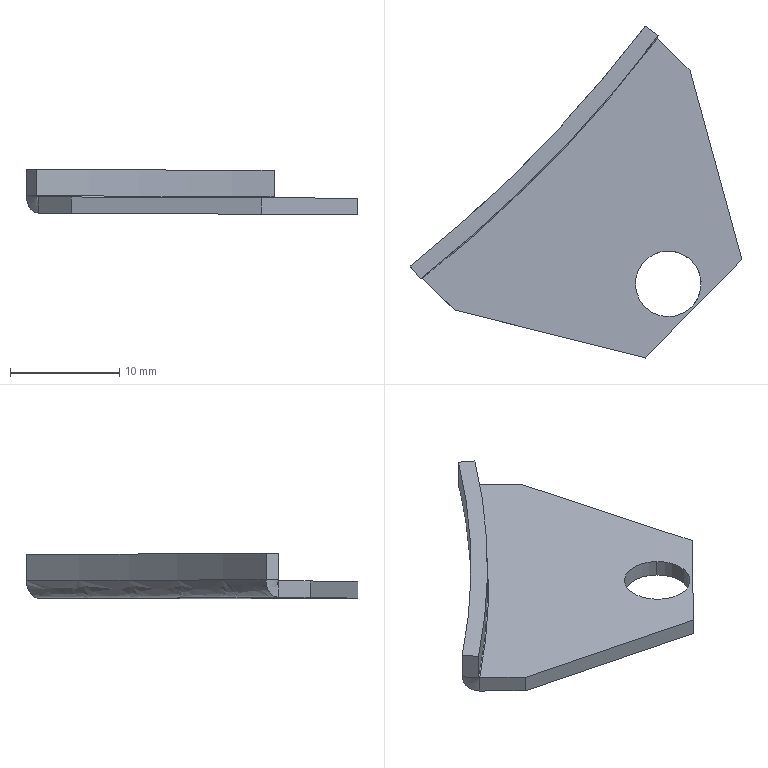Component | SolidWorks | Light-1_LampHolderMountingPlate-11 | 1 solid | 18 faces | box 30.32 x 30.33 x 4.13 mm | volume 795 mm3 | plane 10 | cylinder 4 | spline 4 | commonest cylinder face diameters 6 x2 244.197 x1 247.197 x1
STEP:
#1=CARTESIAN_POINT('',(-209.83,272.853,13.52));
#2=VERTEX_POINT('',#1);
#3=CARTESIAN_POINT('',(-209.665,273.022,13.52));
#4=VERTEX_POINT('',#3);
#5=CARTESIAN_POINT('',(-209.748,272.937,13.52));
#6=DIRECTION('',(0.004294,0.,1.));
#7=DIRECTION('',(-0.6995,-0.7146,0.003003));
#8=AXIS2_PLACEMENT_3D('',#5,#6,#7);
#9=CIRCLE('',#8,0.1181);
#10=EDGE_CURVE('',#2,#4,#9,.T.);
#11=ORIENTED_EDGE('',*,*,#10,.T.);
#12=CARTESIAN_POINT('',(-209.665,273.022,13.461));
#13=VERTEX_POINT('',#12);
#14=CARTESIAN_POINT('',(-209.665,273.022,13.52));
#15=DIRECTION('',(-0.004294,-0.,-1.));
#16=VECTOR('',#15,39.37);
#17=LINE('',#14,#16);
#18=EDGE_CURVE('',#4,#13,#17,.T.);
#19=ORIENTED_EDGE('',*,*,#18,.T.);
#20=CARTESIAN_POINT('',(-209.83,272.853,13.461));
#21=VERTEX_POINT('',#20);
#22=CARTESIAN_POINT('',(-209.748,272.937,13.461));
#23=DIRECTION('',(-0.004294,-0.,-1.));
#24=DIRECTION('',(-0.6995,-0.7146,0.003003));
#25=AXIS2_PLACEMENT_3D('',#22,#23,#24);
#26=CIRCLE('',#25,0.1181);
#27=EDGE_CURVE('',#13,#21,#26,.T.);
#28=ORIENTED_EDGE('',*,*,#27,.T.);
#29=CARTESIAN_POINT('',(-209.83,272.853,13.52));
#30=DIRECTION('',(-0.004294,-0.,-1.));
#31=VECTOR('',#30,39.37);
#32=LINE('',#29,#31);
#33=EDGE_CURVE('',#2,#21,#32,.T.);
#34=ORIENTED_EDGE('',*,*,#33,.F.);
#35=EDGE_LOOP('',(#11,#19,#28,#34));
#36=FACE_OUTER_BOUND('',#35,.T.);
#37=CARTESIAN_POINT('',(-209.748,272.937,13.52));
#38=DIRECTION('',(-0.004294,-0.,-1.));
#39=DIRECTION('',(-0.6995,-0.7146,0.003003));
#40=AXIS2_PLACEMENT_3D('',#37,#38,#39);
#41=CYLINDRICAL_SURFACE('',#40,0.1181);
#42=ADVANCED_FACE('',(#36),#41,.F.);
#43=ORIENTED_EDGE('',*,*,#18,.F.);
#44=CARTESIAN_POINT('',(-209.748,272.937,13.52));
#45=DIRECTION('',(0.004294,0.,1.));
#46=DIRECTION('',(-0.6995,-0.7146,0.003003));
#47=AXIS2_PLACEMENT_3D('',#44,#45,#46);
#48=CIRCLE('',#47,0.1181);
#49=EDGE_CURVE('',#4,#2,#48,.T.);
#50=ORIENTED_EDGE('',*,*,#49,.T.);
#51=ORIENTED_EDGE('',*,*,#33,.T.);
#52=CARTESIAN_POINT('',(-209.748,272.937,13.461));
#53=DIRECTION('',(-0.004294,-0.,-1.));
#54=DIRECTION('',(-0.6995,-0.7146,0.003003));
#55=AXIS2_PLACEMENT_3D('',#52,#53,#54);
#56=CIRCLE('',#55,0.1181);
#57=EDGE_CURVE('',#21,#13,#56,.T.);
#58=ORIENTED_EDGE('',*,*,#57,.T.);
#59=EDGE_LOOP('',(#43,#50,#51,#58));
#60=FACE_OUTER_BOUND('',#59,.T.);
#61=CARTESIAN_POINT('',(-209.748,272.937,13.52));
#62=DIRECTION('',(-0.004294,-0.,-1.));
#63=DIRECTION('',(-0.6995,-0.7146,0.003003));
#64=AXIS2_PLACEMENT_3D('',#61,#62,#63);
#65=CYLINDRICAL_SURFACE('',#64,0.1181);
#66=ADVANCED_FACE('',(#60),#65,.F.);
#67=ORIENTED_EDGE('',*,*,#57,.F.);
#68=ORIENTED_EDGE('',*,*,#27,.F.);
#69=EDGE_LOOP('',(#67,#68));
#70=FACE_BOUND('',#69,.T.);
#71=CARTESIAN_POINT('',(-209.483,273.025,13.46));
#72=VERTEX_POINT('',#71);
#73=CARTESIAN_POINT('',(-209.83,272.671,13.461));
#74=VERTEX_POINT('',#73);
#75=CARTESIAN_POINT('',(-209.657,272.848,13.461));
#76=DIRECTION('',(-0.6995,-0.7146,0.003003));
#77=VECTOR('',#76,39.37);
#78=LINE('',#75,#77);
#79=EDGE_CURVE('',#72,#74,#78,.T.);
#80=ORIENTED_EDGE('',*,*,#79,.T.);
#81=CARTESIAN_POINT('',(-210.515,272.843,13.464));
#82=VERTEX_POINT('',#81);
#83=CARTESIAN_POINT('',(-209.83,272.671,13.461));
#84=DIRECTION('',(-0.9698,0.2438,0.004164));
#85=VECTOR('',#84,39.37);
#86=LINE('',#83,#85);
#87=EDGE_CURVE('',#74,#82,#86,.T.);
#88=ORIENTED_EDGE('',*,*,#87,.T.);
#89=CARTESIAN_POINT('',(-210.631,272.957,13.465));
#90=VERTEX_POINT('',#89);
#91=CARTESIAN_POINT('',(-210.357,272.688,13.464));
#92=DIRECTION('',(-0.7146,0.6995,0.003068));
#93=VECTOR('',#92,39.37);
#94=LINE('',#91,#93);
#95=EDGE_CURVE('',#82,#90,#94,.T.);
#96=ORIENTED_EDGE('',*,*,#95,.T.);
#97=CARTESIAN_POINT('',(-209.786,273.82,13.461));
#98=VERTEX_POINT('',#97);
#99=CARTESIAN_POINT('',(-210.631,272.957,13.465));
#100=CARTESIAN_POINT('',(-210.592,272.988,13.465));
#101=CARTESIAN_POINT('',(-210.553,273.02,13.465));
#102=CARTESIAN_POINT('',(-210.476,273.086,13.464));
#103=CARTESIAN_POINT('',(-210.438,273.119,13.464));
#104=CARTESIAN_POINT('',(-210.326,273.22,13.464));
#105=CARTESIAN_POINT('',(-210.253,273.29,13.463));
#106=CARTESIAN_POINT('',(-210.147,273.399,13.463));
#107=CARTESIAN_POINT('',(-210.095,273.453,13.463));
#108=CARTESIAN_POINT('',(-210.044,273.51,13.462));
#109=CARTESIAN_POINT('',(-210.01,273.547,13.462));
#110=CARTESIAN_POINT('',(-209.993,273.566,13.462));
#111=CARTESIAN_POINT('',(-209.911,273.662,13.462));
#112=CARTESIAN_POINT('',(-209.847,273.74,13.461));
#113=CARTESIAN_POINT('',(-209.786,273.82,13.461));
#114=B_SPLINE_CURVE_WITH_KNOTS('',3,(#99,#100,#101,#102,#103,#104,#105,#106,#107,#108,#109,#110,#111,#112,#113),.UNSPECIFIED.,.F.,.F.,(4,2,2,2,1,2,2,4),(0.,0.125,0.25,0.5,0.625,0.6875,0.75,1.),.UNSPECIFIED.);
#115=EDGE_CURVE('',#90,#98,#114,.T.);
#116=ORIENTED_EDGE('',*,*,#115,.T.);
#117=CARTESIAN_POINT('',(-209.67,273.706,13.461));
#118=VERTEX_POINT('',#117);
#119=CARTESIAN_POINT('',(-209.512,273.552,13.46));
#120=DIRECTION('',(0.7146,-0.6995,-0.003068));
#121=VECTOR('',#120,39.37);
#122=LINE('',#119,#121);
#123=EDGE_CURVE('',#98,#118,#122,.T.);
#124=ORIENTED_EDGE('',*,*,#123,.T.);
#125=CARTESIAN_POINT('',(-209.67,273.706,13.461));
#126=DIRECTION('',(0.2645,-0.9644,-0.001136));
#127=VECTOR('',#126,39.37);
#128=LINE('',#125,#127);
#129=EDGE_CURVE('',#118,#72,#128,.T.);
#130=ORIENTED_EDGE('',*,*,#129,.T.);
#131=EDGE_LOOP('',(#80,#88,#96,#116,#124,#130));
#132=FACE_OUTER_BOUND('',#131,.T.);
#133=CARTESIAN_POINT('',(-209.234,273.28,13.459));
#134=DIRECTION('',(-0.004294,-0.,-1.));
#135=DIRECTION('',(-0.6995,-0.7146,0.003003));
#136=AXIS2_PLACEMENT_3D('',#133,#134,#135);
#137=PLANE('',#136);
#138=ADVANCED_FACE('',(#70,#132),#137,.T.);
#139=ORIENTED_EDGE('',*,*,#10,.F.);
#140=ORIENTED_EDGE('',*,*,#49,.F.);
#141=EDGE_LOOP('',(#139,#140));
#142=FACE_BOUND('',#141,.T.);
#143=CARTESIAN_POINT('',(-210.514,272.843,13.523));
#144=VERTEX_POINT('',#143);
#145=CARTESIAN_POINT('',(-210.631,272.957,13.524));
#146=VERTEX_POINT('',#145);
#147=CARTESIAN_POINT('',(-210.357,272.688,13.523));
#148=DIRECTION('',(-0.7146,0.6995,0.003068));
#149=VECTOR('',#148,39.37);
#150=LINE('',#147,#149);
#151=EDGE_CURVE('',#144,#146,#150,.T.);
#152=ORIENTED_EDGE('',*,*,#151,.F.);
#153=CARTESIAN_POINT('',(-209.83,272.671,13.52));
#154=VERTEX_POINT('',#153);
#155=CARTESIAN_POINT('',(-209.83,272.671,13.52));
#156=DIRECTION('',(-0.9698,0.2438,0.004164));
#157=VECTOR('',#156,39.37);
#158=LINE('',#155,#157);
#159=EDGE_CURVE('',#154,#144,#158,.T.);
#160=ORIENTED_EDGE('',*,*,#159,.F.);
#161=CARTESIAN_POINT('',(-209.483,273.025,13.519));
#162=VERTEX_POINT('',#161);
#163=CARTESIAN_POINT('',(-209.656,272.848,13.52));
#164=DIRECTION('',(-0.6995,-0.7146,0.003003));
#165=VECTOR('',#164,39.37);
#166=LINE('',#163,#165);
#167=EDGE_CURVE('',#162,#154,#166,.T.);
#168=ORIENTED_EDGE('',*,*,#167,.F.);
#169=CARTESIAN_POINT('',(-209.669,273.706,13.52));
#170=VERTEX_POINT('',#169);
#171=CARTESIAN_POINT('',(-209.669,273.706,13.52));
#172=DIRECTION('',(0.2645,-0.9644,-0.001136));
#173=VECTOR('',#172,39.37);
#174=LINE('',#171,#173);
#175=EDGE_CURVE('',#170,#162,#174,.T.);
#176=ORIENTED_EDGE('',*,*,#175,.F.);
#177=CARTESIAN_POINT('',(-209.786,273.82,13.52));
#178=VERTEX_POINT('',#177);
#179=CARTESIAN_POINT('',(-209.512,273.552,13.519));
#180=DIRECTION('',(0.7146,-0.6995,-0.003068));
#181=VECTOR('',#180,39.37);
#182=LINE('',#179,#181);
#183=EDGE_CURVE('',#178,#170,#182,.T.);
#184=ORIENTED_EDGE('',*,*,#183,.F.);
#185=CARTESIAN_POINT('',(-210.631,272.957,13.524));
#186=CARTESIAN_POINT('',(-210.314,273.209,13.523));
#187=CARTESIAN_POINT('',(-210.031,273.498,13.521));
#188=CARTESIAN_POINT('',(-209.786,273.82,13.52));
#189=(BOUNDED_CURVE()B_SPLINE_CURVE(3,(#185,#186,#187,#188),.UNSPECIFIED.,.F.,.F.)B_SPLINE_CURVE_WITH_KNOTS((4,4),(0.,1.),.UNSPECIFIED.)CURVE()GEOMETRIC_REPRESENTATION_ITEM()RATIONAL_B_SPLINE_CURVE((0.9564,0.9515,0.9515,0.9564))REPRESENTATION_ITEM(''));
#190=EDGE_CURVE('',#146,#178,#189,.T.);
#191=ORIENTED_EDGE('',*,*,#190,.F.);
#192=EDGE_LOOP('',(#152,#160,#168,#176,#184,#191));
#193=FACE_OUTER_BOUND('',#192,.T.);
#194=CARTESIAN_POINT('',(-209.234,273.28,13.518));
#195=DIRECTION('',(-0.004294,-0.,-1.));
#196=DIRECTION('',(-0.6995,-0.7146,0.003003));
#197=AXIS2_PLACEMENT_3D('',#194,#195,#196);
#198=PLANE('',#197);
#199=ADVANCED_FACE('',(#142,#193),#198,.F.);
#200=CARTESIAN_POINT('',(-210.515,272.843,13.494));
#201=DIRECTION('',(-0.004294,-0.,-1.));
#202=VECTOR('',#201,39.37);
#203=LINE('',#200,#202);
#204=EDGE_CURVE('',#144,#82,#203,.T.);
#205=ORIENTED_EDGE('',*,*,#204,.T.);
#206=ORIENTED_EDGE('',*,*,#87,.F.);
#207=CARTESIAN_POINT('',(-209.83,272.671,13.491));
#208=DIRECTION('',(0.004294,0.,1.));
#209=VECTOR('',#208,39.37);
#210=LINE('',#207,#209);
#211=EDGE_CURVE('',#74,#154,#210,.T.);
#212=ORIENTED_EDGE('',*,*,#211,.T.);
#213=ORIENTED_EDGE('',*,*,#159,.T.);
#214=EDGE_LOOP('',(#205,#206,#212,#213));
#215=FACE_OUTER_BOUND('',#214,.T.);
#216=CARTESIAN_POINT('',(-209.83,272.671,13.52));
#217=DIRECTION('',(-0.2438,-0.9698,0.001047));
#218=DIRECTION('',(-0.9698,0.2438,0.004164));
#219=AXIS2_PLACEMENT_3D('',#216,#217,#218);
#220=PLANE('',#219);
#221=ADVANCED_FACE('',(#215),#220,.T.);
#222=ORIENTED_EDGE('',*,*,#79,.F.);
#223=CARTESIAN_POINT('',(-209.483,273.025,13.489));
#224=DIRECTION('',(0.004294,0.,1.));
#225=VECTOR('',#224,39.37);
#226=LINE('',#223,#225);
#227=EDGE_CURVE('',#72,#162,#226,.T.);
#228=ORIENTED_EDGE('',*,*,#227,.T.);
#229=ORIENTED_EDGE('',*,*,#167,.T.);
#230=ORIENTED_EDGE('',*,*,#211,.F.);
#231=EDGE_LOOP('',(#222,#228,#229,#230));
#232=FACE_OUTER_BOUND('',#231,.T.);
#233=CARTESIAN_POINT('',(-209.483,273.025,13.519));
#234=DIRECTION('',(0.7146,-0.6995,-0.003068));
#235=DIRECTION('',(-0.6995,-0.7146,0.003003));
#236=AXIS2_PLACEMENT_3D('',#233,#234,#235);
#237=PLANE('',#236);
#238=ADVANCED_FACE('',(#232),#237,.T.);
#239=ORIENTED_EDGE('',*,*,#227,.F.);
#240=ORIENTED_EDGE('',*,*,#129,.F.);
#241=CARTESIAN_POINT('',(-209.67,273.706,13.49));
#242=DIRECTION('',(0.004294,0.,1.));
#243=VECTOR('',#242,39.37);
#244=LINE('',#241,#243);
#245=EDGE_CURVE('',#118,#170,#244,.T.);
#246=ORIENTED_EDGE('',*,*,#245,.T.);
#247=ORIENTED_EDGE('',*,*,#175,.T.);
#248=EDGE_LOOP('',(#239,#240,#246,#247));
#249=FACE_OUTER_BOUND('',#248,.T.);
#250=CARTESIAN_POINT('',(-209.669,273.706,13.52));
#251=DIRECTION('',(0.9644,0.2645,-0.004141));
#252=DIRECTION('',(0.2645,-0.9644,-0.001136));
#253=AXIS2_PLACEMENT_3D('',#250,#251,#252);
#254=PLANE('',#253);
#255=ADVANCED_FACE('',(#249),#254,.T.);
#256=ORIENTED_EDGE('',*,*,#245,.F.);
#257=ORIENTED_EDGE('',*,*,#123,.F.);
#258=CARTESIAN_POINT('',(-209.786,273.82,13.491));
#259=DIRECTION('',(-0.004294,-0.,-1.));
#260=VECTOR('',#259,39.37);
#261=LINE('',#258,#260);
#262=EDGE_CURVE('',#178,#98,#261,.T.);
#263=ORIENTED_EDGE('',*,*,#262,.F.);
#264=ORIENTED_EDGE('',*,*,#183,.T.);
#265=EDGE_LOOP('',(#256,#257,#263,#264));
#266=FACE_OUTER_BOUND('',#265,.T.);
#267=CARTESIAN_POINT('',(-209.786,273.82,13.52));
#268=DIRECTION('',(0.6995,0.7146,-0.003003));
#269=DIRECTION('',(0.7146,-0.6995,-0.003068));
#270=AXIS2_PLACEMENT_3D('',#267,#268,#269);
#271=PLANE('',#270);
#272=ADVANCED_FACE('',(#266),#271,.T.);
#273=ORIENTED_EDGE('',*,*,#115,.F.);
#274=CARTESIAN_POINT('',(-210.677,273.001,13.528));
#275=VERTEX_POINT('',#274);
#276=CARTESIAN_POINT('',(-210.631,272.957,13.465));
#277=CARTESIAN_POINT('',(-210.634,272.96,13.465));
#278=CARTESIAN_POINT('',(-210.637,272.963,13.465));
#279=CARTESIAN_POINT('',(-210.643,272.969,13.467));
#280=CARTESIAN_POINT('',(-210.645,272.972,13.468));
#281=CARTESIAN_POINT('',(-210.651,272.978,13.471));
#282=CARTESIAN_POINT('',(-210.653,272.98,13.473));
#283=CARTESIAN_POINT('',(-210.658,272.985,13.478));
#284=CARTESIAN_POINT('',(-210.66,272.987,13.481));
#285=CARTESIAN_POINT('',(-210.666,272.994,13.489));
#286=CARTESIAN_POINT('',(-210.67,272.997,13.496));
#287=CARTESIAN_POINT('',(-210.675,273.001,13.511));
#288=CARTESIAN_POINT('',(-210.676,273.002,13.52));
#289=CARTESIAN_POINT('',(-210.677,273.001,13.528));
#290=B_SPLINE_CURVE_WITH_KNOTS('',3,(#276,#277,#278,#279,#280,#281,#282,#283,#284,#285,#286,#287,#288,#289),.UNSPECIFIED.,.F.,.F.,(4,2,2,2,2,2,4),(0.,0.0003134,0.0006269,0.0009403,0.001254,0.001881,0.002507),.UNSPECIFIED.);
#291=EDGE_CURVE('',#90,#275,#290,.T.);
#292=ORIENTED_EDGE('',*,*,#291,.T.);
#293=CARTESIAN_POINT('',(-209.832,273.865,13.524));
#294=VERTEX_POINT('',#293);
#295=CARTESIAN_POINT('',(-213.662,276.769,13.541));
#296=DIRECTION('',(0.004294,0.,1.));
#297=DIRECTION('',(0.6199,-0.7847,-0.002662));
#298=AXIS2_PLACEMENT_3D('',#295,#296,#297);
#299=CIRCLE('',#298,4.807);
#300=EDGE_CURVE('',#275,#294,#299,.T.);
#301=ORIENTED_EDGE('',*,*,#300,.T.);
#302=CARTESIAN_POINT('',(-209.832,273.865,13.524));
#303=CARTESIAN_POINT('',(-209.832,273.865,13.52));
#304=CARTESIAN_POINT('',(-209.832,273.864,13.516));
#305=CARTESIAN_POINT('',(-209.831,273.863,13.508));
#306=CARTESIAN_POINT('',(-209.83,273.862,13.504));
#307=CARTESIAN_POINT('',(-209.828,273.859,13.496));
#308=CARTESIAN_POINT('',(-209.827,273.858,13.493));
#309=CARTESIAN_POINT('',(-209.823,273.854,13.486));
#310=CARTESIAN_POINT('',(-209.821,273.853,13.483));
#311=CARTESIAN_POINT('',(-209.815,273.846,13.474));
#312=CARTESIAN_POINT('',(-209.81,273.842,13.469));
#313=CARTESIAN_POINT('',(-209.799,273.831,13.463));
#314=CARTESIAN_POINT('',(-209.793,273.826,13.461));
#315=CARTESIAN_POINT('',(-209.786,273.82,13.461));
#316=B_SPLINE_CURVE_WITH_KNOTS('',3,(#302,#303,#304,#305,#306,#307,#308,#309,#310,#311,#312,#313,#314,#315),.UNSPECIFIED.,.F.,.F.,(4,2,2,2,2,2,4),(0.,0.0003134,0.0006269,0.0009403,0.001254,0.001881,0.002507),.UNSPECIFIED.);
#317=EDGE_CURVE('',#294,#98,#316,.T.);
#318=ORIENTED_EDGE('',*,*,#317,.T.);
#319=EDGE_LOOP('',(#273,#292,#301,#318));
#320=FACE_OUTER_BOUND('',#319,.T.);
#321=CARTESIAN_POINT('',(-210.64,272.943,13.465));
#322=CARTESIAN_POINT('',(-210.313,273.2,13.464));
#323=CARTESIAN_POINT('',(-210.023,273.497,13.463));
#324=CARTESIAN_POINT('',(-209.772,273.829,13.461));
#325=CARTESIAN_POINT('',(-210.666,272.976,13.461));
#326=CARTESIAN_POINT('',(-210.343,273.232,13.46));
#327=CARTESIAN_POINT('',(-210.055,273.526,13.458));
#328=CARTESIAN_POINT('',(-209.806,273.855,13.457));
#329=CARTESIAN_POINT('',(-210.685,273.,13.492));
#330=CARTESIAN_POINT('',(-210.364,273.254,13.49));
#331=CARTESIAN_POINT('',(-210.077,273.546,13.489));
#332=CARTESIAN_POINT('',(-209.83,273.873,13.488));
#333=CARTESIAN_POINT('',(-210.682,272.997,13.534));
#334=CARTESIAN_POINT('',(-210.361,273.251,13.533));
#335=CARTESIAN_POINT('',(-210.074,273.544,13.532));
#336=CARTESIAN_POINT('',(-209.827,273.87,13.531));
#337=(BOUNDED_SURFACE()B_SPLINE_SURFACE(3,3,((#321,#322,#323,#324),(#325,#326,#327,#328),(#329,#330,#331,#332),(#333,#334,#335,#336)),.UNSPECIFIED.,.F.,.F.,.T.)B_SPLINE_SURFACE_WITH_KNOTS((4,4),(4,4),(0.,1.),(0.,1.),.UNSPECIFIED.)GEOMETRIC_REPRESENTATION_ITEM()RATIONAL_B_SPLINE_SURFACE(((1.,0.9946,0.9946,1.),(0.7553,0.7512,0.7512,0.7553),(0.7553,0.7512,0.7512,0.7553),(1.,0.9946,0.9946,1.)))REPRESENTATION_ITEM('')SURFACE());
#338=ADVANCED_FACE('',(#320),#337,.T.);
#339=ORIENTED_EDGE('',*,*,#95,.F.);
#340=ORIENTED_EDGE('',*,*,#204,.F.);
#341=ORIENTED_EDGE('',*,*,#151,.T.);
#342=CARTESIAN_POINT('',(-210.631,272.957,13.494));
#343=DIRECTION('',(-0.004294,-0.,-1.));
#344=VECTOR('',#343,39.37);
#345=LINE('',#342,#344);
#346=EDGE_CURVE('',#146,#90,#345,.T.);
#347=ORIENTED_EDGE('',*,*,#346,.T.);
#348=EDGE_LOOP('',(#339,#340,#341,#347));
#349=FACE_OUTER_BOUND('',#348,.T.);
#350=CARTESIAN_POINT('',(-210.514,272.843,13.523));
#351=DIRECTION('',(-0.6995,-0.7146,0.003003));
#352=DIRECTION('',(-0.7146,0.6995,0.003068));
#353=AXIS2_PLACEMENT_3D('',#350,#351,#352);
#354=PLANE('',#353);
#355=ADVANCED_FACE('',(#349),#354,.T.);
#356=CARTESIAN_POINT('',(-210.64,272.955,13.528));
#357=VERTEX_POINT('',#356);
#358=CARTESIAN_POINT('',(-210.631,272.957,13.524));
#359=CARTESIAN_POINT('',(-210.633,272.957,13.524));
#360=CARTESIAN_POINT('',(-210.635,272.957,13.524));
#361=CARTESIAN_POINT('',(-210.638,272.956,13.526));
#362=CARTESIAN_POINT('',(-210.639,272.956,13.527));
#363=CARTESIAN_POINT('',(-210.64,272.955,13.528));
#364=B_SPLINE_CURVE_WITH_KNOTS('',3,(#358,#359,#360,#361,#362,#363),.UNSPECIFIED.,.F.,.F.,(4,2,4),(0.,0.0001276,0.0002551),.UNSPECIFIED.);
#365=EDGE_CURVE('',#146,#357,#364,.T.);
#366=ORIENTED_EDGE('',*,*,#365,.F.);
#367=ORIENTED_EDGE('',*,*,#190,.T.);
#368=CARTESIAN_POINT('',(-209.784,273.829,13.524));
#369=VERTEX_POINT('',#368);
#370=CARTESIAN_POINT('',(-209.784,273.829,13.524));
#371=CARTESIAN_POINT('',(-209.785,273.828,13.523));
#372=CARTESIAN_POINT('',(-209.786,273.827,13.522));
#373=CARTESIAN_POINT('',(-209.786,273.824,13.521));
#374=CARTESIAN_POINT('',(-209.786,273.822,13.52));
#375=CARTESIAN_POINT('',(-209.786,273.82,13.52));
#376=B_SPLINE_CURVE_WITH_KNOTS('',3,(#370,#371,#372,#373,#374,#375),.UNSPECIFIED.,.F.,.F.,(4,2,4),(0.,0.0001275,0.0002551),.UNSPECIFIED.);
#377=EDGE_CURVE('',#369,#178,#376,.T.);
#378=ORIENTED_EDGE('',*,*,#377,.F.);
#379=CARTESIAN_POINT('',(-213.662,276.769,13.541));
#380=DIRECTION('',(0.004294,0.,1.));
#381=DIRECTION('',(0.6199,-0.7847,-0.002662));
#382=AXIS2_PLACEMENT_3D('',#379,#380,#381);
#383=CIRCLE('',#382,4.866);
#384=EDGE_CURVE('',#357,#369,#383,.T.);
#385=ORIENTED_EDGE('',*,*,#384,.F.);
#386=EDGE_LOOP('',(#366,#367,#378,#385));
#387=FACE_OUTER_BOUND('',#386,.T.);
#388=CARTESIAN_POINT('',(-210.643,272.947,13.524));
#389=CARTESIAN_POINT('',(-210.317,273.205,13.523));
#390=CARTESIAN_POINT('',(-210.027,273.501,13.521));
#391=CARTESIAN_POINT('',(-209.777,273.832,13.52));
#392=CARTESIAN_POINT('',(-210.645,272.949,13.524));
#393=CARTESIAN_POINT('',(-210.319,273.206,13.522));
#394=CARTESIAN_POINT('',(-210.029,273.503,13.521));
#395=CARTESIAN_POINT('',(-209.779,273.834,13.52));
#396=CARTESIAN_POINT('',(-210.646,272.951,13.526));
#397=CARTESIAN_POINT('',(-210.32,273.208,13.524));
#398=CARTESIAN_POINT('',(-210.03,273.504,13.523));
#399=CARTESIAN_POINT('',(-209.78,273.835,13.522));
#400=CARTESIAN_POINT('',(-210.646,272.951,13.528));
#401=CARTESIAN_POINT('',(-210.32,273.208,13.527));
#402=CARTESIAN_POINT('',(-210.03,273.504,13.526));
#403=CARTESIAN_POINT('',(-209.78,273.835,13.525));
#404=(BOUNDED_SURFACE()B_SPLINE_SURFACE(3,3,((#388,#389,#390,#391),(#392,#393,#394,#395),(#396,#397,#398,#399),(#400,#401,#402,#403)),.UNSPECIFIED.,.F.,.F.,.F.)B_SPLINE_SURFACE_WITH_KNOTS((4,4),(4,4),(0.,1.),(0.,1.),.UNSPECIFIED.)GEOMETRIC_REPRESENTATION_ITEM()RATIONAL_B_SPLINE_SURFACE(((1.,0.9946,0.9946,1.),(0.7553,0.7512,0.7512,0.7553),(0.7553,0.7512,0.7512,0.7553),(1.,0.9946,0.9946,1.)))REPRESENTATION_ITEM('')SURFACE());
#405=ADVANCED_FACE('',(#387),#404,.F.);
#406=CARTESIAN_POINT('',(-210.658,272.978,13.528));
#407=DIRECTION('',(-0.6211,0.7837,0.002667));
#408=VECTOR('',#407,39.37);
#409=LINE('',#406,#408);
#410=EDGE_CURVE('',#357,#275,#409,.T.);
#411=ORIENTED_EDGE('',*,*,#410,.T.);
#412=ORIENTED_EDGE('',*,*,#291,.F.);
#413=ORIENTED_EDGE('',*,*,#346,.F.);
#414=ORIENTED_EDGE('',*,*,#365,.T.);
#415=EDGE_LOOP('',(#411,#412,#413,#414));
#416=FACE_OUTER_BOUND('',#415,.T.);
#417=CARTESIAN_POINT('',(-210.631,272.957,13.464));
#418=CARTESIAN_POINT('',(-210.634,272.96,13.464));
#419=CARTESIAN_POINT('',(-210.637,272.964,13.465));
#420=CARTESIAN_POINT('',(-210.642,272.968,13.466));
#421=CARTESIAN_POINT('',(-210.643,272.97,13.467));
#422=CARTESIAN_POINT('',(-210.645,272.972,13.468));
#423=CARTESIAN_POINT('',(-210.646,272.973,13.468));
#424=CARTESIAN_POINT('',(-210.647,272.974,13.469));
#425=CARTESIAN_POINT('',(-210.648,272.974,13.469));
#426=CARTESIAN_POINT('',(-210.648,272.975,13.469));
#427=CARTESIAN_POINT('',(-210.648,272.975,13.469));
#428=CARTESIAN_POINT('',(-210.649,272.975,13.469));
#429=CARTESIAN_POINT('',(-210.649,272.976,13.47));
#430=CARTESIAN_POINT('',(-210.649,272.976,13.47));
#431=CARTESIAN_POINT('',(-210.649,272.976,13.47));
#432=CARTESIAN_POINT('',(-210.65,272.977,13.471));
#433=CARTESIAN_POINT('',(-210.652,272.98,13.472));
#434=CARTESIAN_POINT('',(-210.656,272.983,13.475));
#435=CARTESIAN_POINT('',(-210.657,272.984,13.477));
#436=CARTESIAN_POINT('',(-210.659,272.986,13.479));
#437=CARTESIAN_POINT('',(-210.66,272.987,13.48));
#438=CARTESIAN_POINT('',(-210.661,272.988,13.481));
#439=CARTESIAN_POINT('',(-210.661,272.988,13.481));
#440=CARTESIAN_POINT('',(-210.662,272.989,13.482));
#441=CARTESIAN_POINT('',(-210.662,272.989,13.482));
#442=CARTESIAN_POINT('',(-210.662,272.99,13.483));
#443=CARTESIAN_POINT('',(-210.662,272.99,13.483));
#444=CARTESIAN_POINT('',(-210.665,272.992,13.486));
#445=CARTESIAN_POINT('',(-210.667,272.994,13.49));
#446=CARTESIAN_POINT('',(-210.669,272.996,13.495));
#447=CARTESIAN_POINT('',(-210.67,272.997,13.496));
#448=CARTESIAN_POINT('',(-210.671,272.998,13.499));
#449=CARTESIAN_POINT('',(-210.671,272.998,13.5));
#450=CARTESIAN_POINT('',(-210.672,272.998,13.501));
#451=CARTESIAN_POINT('',(-210.672,272.999,13.501));
#452=CARTESIAN_POINT('',(-210.672,272.999,13.502));
#453=CARTESIAN_POINT('',(-210.672,272.999,13.502));
#454=CARTESIAN_POINT('',(-210.672,272.999,13.502));
#455=CARTESIAN_POINT('',(-210.672,272.999,13.502));
#456=CARTESIAN_POINT('',(-210.672,272.999,13.502));
#457=CARTESIAN_POINT('',(-210.672,272.999,13.502));
#458=CARTESIAN_POINT('',(-210.675,273.001,13.511));
#459=CARTESIAN_POINT('',(-210.676,273.002,13.519));
#460=CARTESIAN_POINT('',(-210.677,273.002,13.528));
#461=CARTESIAN_POINT('',(-210.631,272.957,13.465));
#462=CARTESIAN_POINT('',(-210.634,272.96,13.465));
#463=CARTESIAN_POINT('',(-210.637,272.963,13.465));
#464=CARTESIAN_POINT('',(-210.642,272.968,13.467));
#465=CARTESIAN_POINT('',(-210.643,272.97,13.467));
#466=CARTESIAN_POINT('',(-210.645,272.972,13.468));
#467=CARTESIAN_POINT('',(-210.646,272.973,13.469));
#468=CARTESIAN_POINT('',(-210.647,272.974,13.469));
#469=CARTESIAN_POINT('',(-210.647,272.974,13.469));
#470=CARTESIAN_POINT('',(-210.648,272.975,13.47));
#471=CARTESIAN_POINT('',(-210.648,272.975,13.47));
#472=CARTESIAN_POINT('',(-210.648,272.975,13.47));
#473=CARTESIAN_POINT('',(-210.648,272.975,13.47));
#474=CARTESIAN_POINT('',(-210.649,272.976,13.47));
#475=CARTESIAN_POINT('',(-210.649,272.976,13.47));
#476=CARTESIAN_POINT('',(-210.65,272.977,13.471));
#477=CARTESIAN_POINT('',(-210.652,272.979,13.473));
#478=CARTESIAN_POINT('',(-210.656,272.983,13.476));
#479=CARTESIAN_POINT('',(-210.657,272.984,13.477));
#480=CARTESIAN_POINT('',(-210.659,272.986,13.479));
#481=CARTESIAN_POINT('',(-210.66,272.987,13.48));
#482=CARTESIAN_POINT('',(-210.661,272.988,13.481));
#483=CARTESIAN_POINT('',(-210.661,272.988,13.482));
#484=CARTESIAN_POINT('',(-210.661,272.989,13.482));
#485=CARTESIAN_POINT('',(-210.662,272.989,13.483));
#486=CARTESIAN_POINT('',(-210.662,272.989,13.483));
#487=CARTESIAN_POINT('',(-210.662,272.989,13.483));
#488=CARTESIAN_POINT('',(-210.665,272.992,13.487));
#489=CARTESIAN_POINT('',(-210.667,272.994,13.49));
#490=CARTESIAN_POINT('',(-210.669,272.996,13.495));
#491=CARTESIAN_POINT('',(-210.67,272.997,13.497));
#492=CARTESIAN_POINT('',(-210.67,272.997,13.499));
#493=CARTESIAN_POINT('',(-210.671,272.998,13.5));
#494=CARTESIAN_POINT('',(-210.671,272.998,13.501));
#495=CARTESIAN_POINT('',(-210.671,272.998,13.501));
#496=CARTESIAN_POINT('',(-210.672,272.998,13.502));
#497=CARTESIAN_POINT('',(-210.672,272.998,13.502));
#498=CARTESIAN_POINT('',(-210.672,272.998,13.502));
#499=CARTESIAN_POINT('',(-210.672,272.998,13.502));
#500=CARTESIAN_POINT('',(-210.672,272.998,13.503));
#501=CARTESIAN_POINT('',(-210.672,272.998,13.503));
#502=CARTESIAN_POINT('',(-210.674,273.001,13.511));
#503=CARTESIAN_POINT('',(-210.676,273.002,13.519));
#504=CARTESIAN_POINT('',(-210.677,273.001,13.528));
#505=CARTESIAN_POINT('',(-210.631,272.957,13.524));
#506=CARTESIAN_POINT('',(-210.632,272.957,13.524));
#507=CARTESIAN_POINT('',(-210.632,272.957,13.524));
#508=CARTESIAN_POINT('',(-210.633,272.957,13.524));
#509=CARTESIAN_POINT('',(-210.633,272.957,13.524));
#510=CARTESIAN_POINT('',(-210.633,272.957,13.524));
#511=CARTESIAN_POINT('',(-210.633,272.957,13.524));
#512=CARTESIAN_POINT('',(-210.633,272.957,13.524));
#513=CARTESIAN_POINT('',(-210.634,272.957,13.524));
#514=CARTESIAN_POINT('',(-210.634,272.957,13.524));
#515=CARTESIAN_POINT('',(-210.634,272.957,13.524));
#516=CARTESIAN_POINT('',(-210.634,272.957,13.524));
#517=CARTESIAN_POINT('',(-210.634,272.957,13.524));
#518=CARTESIAN_POINT('',(-210.634,272.957,13.524));
#519=CARTESIAN_POINT('',(-210.634,272.957,13.524));
#520=CARTESIAN_POINT('',(-210.634,272.957,13.524));
#521=CARTESIAN_POINT('',(-210.634,272.957,13.524));
#522=CARTESIAN_POINT('',(-210.635,272.957,13.525));
#523=CARTESIAN_POINT('',(-210.635,272.957,13.525));
#524=CARTESIAN_POINT('',(-210.635,272.957,13.525));
#525=CARTESIAN_POINT('',(-210.636,272.957,13.525));
#526=CARTESIAN_POINT('',(-210.636,272.957,13.525));
#527=CARTESIAN_POINT('',(-210.636,272.957,13.525));
#528=CARTESIAN_POINT('',(-210.636,272.957,13.525));
#529=CARTESIAN_POINT('',(-210.636,272.957,13.525));
#530=CARTESIAN_POINT('',(-210.636,272.957,13.525));
#531=CARTESIAN_POINT('',(-210.636,272.957,13.525));
#532=CARTESIAN_POINT('',(-210.636,272.957,13.525));
#533=CARTESIAN_POINT('',(-210.637,272.957,13.526));
#534=CARTESIAN_POINT('',(-210.637,272.956,13.526));
#535=CARTESIAN_POINT('',(-210.638,272.956,13.526));
#536=CARTESIAN_POINT('',(-210.638,272.956,13.526));
#537=CARTESIAN_POINT('',(-210.638,272.956,13.526));
#538=CARTESIAN_POINT('',(-210.638,272.956,13.526));
#539=CARTESIAN_POINT('',(-210.638,272.956,13.526));
#540=CARTESIAN_POINT('',(-210.638,272.956,13.526));
#541=CARTESIAN_POINT('',(-210.638,272.956,13.526));
#542=CARTESIAN_POINT('',(-210.638,272.956,13.526));
#543=CARTESIAN_POINT('',(-210.638,272.956,13.526));
#544=CARTESIAN_POINT('',(-210.638,272.956,13.526));
#545=CARTESIAN_POINT('',(-210.638,272.956,13.526));
#546=CARTESIAN_POINT('',(-210.639,272.956,13.527));
#547=CARTESIAN_POINT('',(-210.639,272.956,13.527));
#548=CARTESIAN_POINT('',(-210.64,272.955,13.528));
#549=CARTESIAN_POINT('',(-210.631,272.957,13.525));
#550=CARTESIAN_POINT('',(-210.632,272.957,13.525));
#551=CARTESIAN_POINT('',(-210.632,272.957,13.525));
#552=CARTESIAN_POINT('',(-210.633,272.957,13.525));
#553=CARTESIAN_POINT('',(-210.633,272.957,13.525));
#554=CARTESIAN_POINT('',(-210.633,272.957,13.525));
#555=CARTESIAN_POINT('',(-210.633,272.957,13.525));
#556=CARTESIAN_POINT('',(-210.633,272.957,13.525));
#557=CARTESIAN_POINT('',(-210.633,272.957,13.525));
#558=CARTESIAN_POINT('',(-210.633,272.957,13.525));
#559=CARTESIAN_POINT('',(-210.633,272.957,13.525));
#560=CARTESIAN_POINT('',(-210.634,272.957,13.525));
#561=CARTESIAN_POINT('',(-210.634,272.957,13.525));
#562=CARTESIAN_POINT('',(-210.634,272.957,13.525));
#563=CARTESIAN_POINT('',(-210.634,272.957,13.525));
#564=CARTESIAN_POINT('',(-210.634,272.957,13.525));
#565=CARTESIAN_POINT('',(-210.634,272.957,13.525));
#566=CARTESIAN_POINT('',(-210.635,272.957,13.525));
#567=CARTESIAN_POINT('',(-210.635,272.957,13.525));
#568=CARTESIAN_POINT('',(-210.635,272.957,13.525));
#569=CARTESIAN_POINT('',(-210.635,272.957,13.525));
#570=CARTESIAN_POINT('',(-210.635,272.956,13.525));
#571=CARTESIAN_POINT('',(-210.636,272.956,13.525));
#572=CARTESIAN_POINT('',(-210.636,272.956,13.525));
#573=CARTESIAN_POINT('',(-210.636,272.956,13.525));
#574=CARTESIAN_POINT('',(-210.636,272.956,13.525));
#575=CARTESIAN_POINT('',(-210.636,272.956,13.525));
#576=CARTESIAN_POINT('',(-210.636,272.956,13.526));
#577=CARTESIAN_POINT('',(-210.637,272.956,13.526));
#578=CARTESIAN_POINT('',(-210.637,272.956,13.526));
#579=CARTESIAN_POINT('',(-210.637,272.956,13.526));
#580=CARTESIAN_POINT('',(-210.637,272.956,13.526));
#581=CARTESIAN_POINT('',(-210.638,272.956,13.526));
#582=CARTESIAN_POINT('',(-210.638,272.956,13.526));
#583=CARTESIAN_POINT('',(-210.638,272.956,13.526));
#584=CARTESIAN_POINT('',(-210.638,272.956,13.526));
#585=CARTESIAN_POINT('',(-210.638,272.956,13.526));
#586=CARTESIAN_POINT('',(-210.638,272.956,13.527));
#587=CARTESIAN_POINT('',(-210.638,272.956,13.527));
#588=CARTESIAN_POINT('',(-210.638,272.956,13.527));
#589=CARTESIAN_POINT('',(-210.638,272.956,13.527));
#590=CARTESIAN_POINT('',(-210.638,272.955,13.527));
#591=CARTESIAN_POINT('',(-210.639,272.955,13.527));
#592=CARTESIAN_POINT('',(-210.639,272.955,13.528));
#593=B_SPLINE_SURFACE_WITH_KNOTS('',1,3,((#417,#418,#419,#420,#421,#422,#423,#424,#425,#426,#427,#428,#429,#430,#431,#432,#433,#434,#435,#436,#437,#438,#439,#440,#441,#442,#443,#444,#445,#446,#447,#448,#449,#450,#451,#452,#453,#454,#455,#456,#457,#458,#459,#460),(#461,#462,#463,#464,#465,#466,#467,#468,#469,#470,#471,#472,#473,#474,#475,#476,#477,#478,#479,#480,#481,#482,#483,#484,#485,#486,#487,#488,#489,#490,#491,#492,#493,#494,#495,#496,#497,#498,#499,#500,#501,#502,#503,#504),(#505,#506,#507,#508,#509,#510,#511,#512,#513,#514,#515,#516,#517,#518,#519,#520,#521,#522,#523,#524,#525,#526,#527,#528,#529,#530,#531,#532,#533,#534,#535,#536,#537,#538,#539,#540,#541,#542,#543,#544,#545,#546,#547,#548),(#549,#550,#551,#552,#553,#554,#555,#556,#557,#558,#559,#560,#561,#562,#563,#564,#565,#566,#567,#568,#569,#570,#571,#572,#573,#574,#575,#576,#577,#578,#579,#580,#581,#582,#583,#584,#585,#586,#587,#588,#589,#590,#591,#592)),.UNSPECIFIED.,.F.,.F.,.F.,(2,1,1,2),(4,2,2,2,2,2,2,2,2,2,2,2,2,2,2,2,2,2,2,2,2,4),(-0.01,0.,1.,1.01),(0.,0.125,0.1875,0.2188,0.2344,0.2422,0.2461,0.25,0.375,0.4375,0.4688,0.4844,0.4922,0.5,0.625,0.6875,0.7188,0.7344,0.7422,0.7461,0.75,1.),.UNSPECIFIED.);
#594=ADVANCED_FACE('',(#416),#593,.T.);
#595=ORIENTED_EDGE('',*,*,#262,.T.);
#596=ORIENTED_EDGE('',*,*,#317,.F.);
#597=CARTESIAN_POINT('',(-209.808,273.847,13.524));
#598=DIRECTION('',(-0.7969,0.6041,0.003422));
#599=VECTOR('',#598,39.37);
#600=LINE('',#597,#599);
#601=EDGE_CURVE('',#369,#294,#600,.T.);
#602=ORIENTED_EDGE('',*,*,#601,.F.);
#603=ORIENTED_EDGE('',*,*,#377,.T.);
#604=EDGE_LOOP('',(#595,#596,#602,#603));
#605=FACE_OUTER_BOUND('',#604,.T.);
#606=CARTESIAN_POINT('',(-209.832,273.865,13.525));
#607=CARTESIAN_POINT('',(-209.832,273.865,13.525));
#608=CARTESIAN_POINT('',(-209.832,273.865,13.525));
#609=CARTESIAN_POINT('',(-209.832,273.865,13.524));
#610=CARTESIAN_POINT('',(-209.832,273.865,13.52));
#611=CARTESIAN_POINT('',(-209.832,273.864,13.516));
#612=CARTESIAN_POINT('',(-209.831,273.863,13.509));
#613=CARTESIAN_POINT('',(-209.831,273.863,13.507));
#614=CARTESIAN_POINT('',(-209.83,273.862,13.504));
#615=CARTESIAN_POINT('',(-209.83,273.862,13.503));
#616=CARTESIAN_POINT('',(-209.83,273.861,13.501));
#617=CARTESIAN_POINT('',(-209.83,273.861,13.501));
#618=CARTESIAN_POINT('',(-209.829,273.861,13.5));
#619=CARTESIAN_POINT('',(-209.829,273.861,13.5));
#620=CARTESIAN_POINT('',(-209.829,273.861,13.5));
#621=CARTESIAN_POINT('',(-209.829,273.861,13.499));
#622=CARTESIAN_POINT('',(-209.829,273.86,13.499));
#623=CARTESIAN_POINT('',(-209.829,273.86,13.499));
#624=CARTESIAN_POINT('',(-209.829,273.86,13.499));
#625=CARTESIAN_POINT('',(-209.829,273.86,13.499));
#626=CARTESIAN_POINT('',(-209.828,273.86,13.497));
#627=CARTESIAN_POINT('',(-209.828,273.859,13.494));
#628=CARTESIAN_POINT('',(-209.825,273.856,13.489));
#629=CARTESIAN_POINT('',(-209.825,273.856,13.487));
#630=CARTESIAN_POINT('',(-209.823,273.854,13.484));
#631=CARTESIAN_POINT('',(-209.822,273.853,13.484));
#632=CARTESIAN_POINT('',(-209.822,273.852,13.482));
#633=CARTESIAN_POINT('',(-209.821,273.852,13.482));
#634=CARTESIAN_POINT('',(-209.821,273.852,13.481));
#635=CARTESIAN_POINT('',(-209.821,273.851,13.481));
#636=CARTESIAN_POINT('',(-209.82,273.851,13.48));
#637=CARTESIAN_POINT('',(-209.82,273.851,13.48));
#638=CARTESIAN_POINT('',(-209.82,273.851,13.48));
#639=CARTESIAN_POINT('',(-209.82,273.851,13.48));
#640=CARTESIAN_POINT('',(-209.818,273.849,13.476));
#641=CARTESIAN_POINT('',(-209.815,273.846,13.474));
#642=CARTESIAN_POINT('',(-209.811,273.843,13.47));
#643=CARTESIAN_POINT('',(-209.81,273.842,13.469));
#644=CARTESIAN_POINT('',(-209.809,273.84,13.468));
#645=CARTESIAN_POINT('',(-209.808,273.84,13.468));
#646=CARTESIAN_POINT('',(-209.807,273.839,13.467));
#647=CARTESIAN_POINT('',(-209.807,273.839,13.467));
#648=CARTESIAN_POINT('',(-209.806,273.838,13.467));
#649=CARTESIAN_POINT('',(-209.806,273.838,13.466));
#650=CARTESIAN_POINT('',(-209.806,273.838,13.466));
#651=CARTESIAN_POINT('',(-209.806,273.838,13.466));
#652=CARTESIAN_POINT('',(-209.8,273.832,13.463));
#653=CARTESIAN_POINT('',(-209.793,273.826,13.461));
#654=CARTESIAN_POINT('',(-209.786,273.82,13.461));
#655=CARTESIAN_POINT('',(-209.831,273.865,13.525));
#656=CARTESIAN_POINT('',(-209.831,273.865,13.525));
#657=CARTESIAN_POINT('',(-209.831,273.865,13.525));
#658=CARTESIAN_POINT('',(-209.832,273.865,13.524));
#659=CARTESIAN_POINT('',(-209.832,273.865,13.52));
#660=CARTESIAN_POINT('',(-209.832,273.864,13.516));
#661=CARTESIAN_POINT('',(-209.831,273.863,13.509));
#662=CARTESIAN_POINT('',(-209.831,273.862,13.507));
#663=CARTESIAN_POINT('',(-209.83,273.862,13.504));
#664=CARTESIAN_POINT('',(-209.83,273.861,13.503));
#665=CARTESIAN_POINT('',(-209.829,273.861,13.502));
#666=CARTESIAN_POINT('',(-209.829,273.861,13.501));
#667=CARTESIAN_POINT('',(-209.829,273.86,13.5));
#668=CARTESIAN_POINT('',(-209.829,273.86,13.5));
#669=CARTESIAN_POINT('',(-209.829,273.86,13.5));
#670=CARTESIAN_POINT('',(-209.829,273.86,13.5));
#671=CARTESIAN_POINT('',(-209.829,273.86,13.499));
#672=CARTESIAN_POINT('',(-209.829,273.86,13.499));
#673=CARTESIAN_POINT('',(-209.829,273.86,13.499));
#674=CARTESIAN_POINT('',(-209.829,273.86,13.499));
#675=CARTESIAN_POINT('',(-209.828,273.859,13.497));
#676=CARTESIAN_POINT('',(-209.827,273.858,13.494));
#677=CARTESIAN_POINT('',(-209.825,273.856,13.489));
#678=CARTESIAN_POINT('',(-209.824,273.855,13.488));
#679=CARTESIAN_POINT('',(-209.823,273.854,13.485));
#680=CARTESIAN_POINT('',(-209.822,273.853,13.484));
#681=CARTESIAN_POINT('',(-209.821,273.852,13.482));
#682=CARTESIAN_POINT('',(-209.821,273.852,13.482));
#683=CARTESIAN_POINT('',(-209.82,273.851,13.481));
#684=CARTESIAN_POINT('',(-209.82,273.851,13.481));
#685=CARTESIAN_POINT('',(-209.82,273.851,13.481));
#686=CARTESIAN_POINT('',(-209.82,273.851,13.48));
#687=CARTESIAN_POINT('',(-209.82,273.851,13.48));
#688=CARTESIAN_POINT('',(-209.82,273.851,13.48));
#689=CARTESIAN_POINT('',(-209.817,273.848,13.477));
#690=CARTESIAN_POINT('',(-209.815,273.846,13.474));
#691=CARTESIAN_POINT('',(-209.811,273.843,13.471));
#692=CARTESIAN_POINT('',(-209.81,273.842,13.47));
#693=CARTESIAN_POINT('',(-209.808,273.84,13.469));
#694=CARTESIAN_POINT('',(-209.808,273.839,13.468));
#695=CARTESIAN_POINT('',(-209.807,273.839,13.468));
#696=CARTESIAN_POINT('',(-209.807,273.838,13.467));
#697=CARTESIAN_POINT('',(-209.806,273.838,13.467));
#698=CARTESIAN_POINT('',(-209.806,273.838,13.467));
#699=CARTESIAN_POINT('',(-209.806,273.838,13.467));
#700=CARTESIAN_POINT('',(-209.806,273.838,13.467));
#701=CARTESIAN_POINT('',(-209.8,273.832,13.463));
#702=CARTESIAN_POINT('',(-209.793,273.826,13.461));
#703=CARTESIAN_POINT('',(-209.786,273.82,13.461));
#704=CARTESIAN_POINT('',(-209.784,273.829,13.524));
#705=CARTESIAN_POINT('',(-209.784,273.829,13.524));
#706=CARTESIAN_POINT('',(-209.784,273.829,13.524));
#707=CARTESIAN_POINT('',(-209.784,273.829,13.524));
#708=CARTESIAN_POINT('',(-209.785,273.829,13.524));
#709=CARTESIAN_POINT('',(-209.785,273.829,13.524));
#710=CARTESIAN_POINT('',(-209.785,273.828,13.523));
#711=CARTESIAN_POINT('',(-209.785,273.828,13.523));
#712=CARTESIAN_POINT('',(-209.785,273.828,13.523));
#713=CARTESIAN_POINT('',(-209.785,273.828,13.523));
#714=CARTESIAN_POINT('',(-209.785,273.828,13.523));
#715=CARTESIAN_POINT('',(-209.785,273.827,13.523));
#716=CARTESIAN_POINT('',(-209.785,273.827,13.523));
#717=CARTESIAN_POINT('',(-209.785,273.827,13.523));
#718=CARTESIAN_POINT('',(-209.785,273.827,13.523));
#719=CARTESIAN_POINT('',(-209.785,273.827,13.523));
#720=CARTESIAN_POINT('',(-209.785,273.827,13.523));
#721=CARTESIAN_POINT('',(-209.785,273.827,13.523));
#722=CARTESIAN_POINT('',(-209.785,273.827,13.523));
#723=CARTESIAN_POINT('',(-209.785,273.827,13.523));
#724=CARTESIAN_POINT('',(-209.785,273.827,13.523));
#725=CARTESIAN_POINT('',(-209.786,273.827,13.522));
#726=CARTESIAN_POINT('',(-209.786,273.826,13.522));
#727=CARTESIAN_POINT('',(-209.786,273.826,13.522));
#728=CARTESIAN_POINT('',(-209.786,273.826,13.522));
#729=CARTESIAN_POINT('',(-209.786,273.826,13.522));
#730=CARTESIAN_POINT('',(-209.786,273.826,13.522));
#731=CARTESIAN_POINT('',(-209.786,273.826,13.522));
#732=CARTESIAN_POINT('',(-209.786,273.825,13.522));
#733=CARTESIAN_POINT('',(-209.786,273.825,13.522));
#734=CARTESIAN_POINT('',(-209.786,273.825,13.521));
#735=CARTESIAN_POINT('',(-209.786,273.825,13.521));
#736=CARTESIAN_POINT('',(-209.786,273.825,13.521));
#737=CARTESIAN_POINT('',(-209.786,273.825,13.521));
#738=CARTESIAN_POINT('',(-209.786,273.825,13.521));
#739=CARTESIAN_POINT('',(-209.786,273.824,13.521));
#740=CARTESIAN_POINT('',(-209.786,273.824,13.521));
#741=CARTESIAN_POINT('',(-209.786,273.824,13.521));
#742=CARTESIAN_POINT('',(-209.786,273.823,13.521));
#743=CARTESIAN_POINT('',(-209.786,273.823,13.521));
#744=CARTESIAN_POINT('',(-209.786,273.823,13.521));
#745=CARTESIAN_POINT('',(-209.786,273.823,13.521));
#746=CARTESIAN_POINT('',(-209.786,273.823,13.521));
#747=CARTESIAN_POINT('',(-209.786,273.823,13.521));
#748=CARTESIAN_POINT('',(-209.786,273.823,13.521));
#749=CARTESIAN_POINT('',(-209.786,273.823,13.521));
#750=CARTESIAN_POINT('',(-209.786,273.822,13.52));
#751=CARTESIAN_POINT('',(-209.786,273.821,13.52));
#752=CARTESIAN_POINT('',(-209.786,273.82,13.52));
#753=CARTESIAN_POINT('',(-209.784,273.829,13.524));
#754=CARTESIAN_POINT('',(-209.784,273.829,13.524));
#755=CARTESIAN_POINT('',(-209.784,273.829,13.524));
#756=CARTESIAN_POINT('',(-209.784,273.829,13.524));
#757=CARTESIAN_POINT('',(-209.784,273.828,13.524));
#758=CARTESIAN_POINT('',(-209.784,273.828,13.524));
#759=CARTESIAN_POINT('',(-209.785,273.828,13.523));
#760=CARTESIAN_POINT('',(-209.785,273.828,13.523));
#761=CARTESIAN_POINT('',(-209.785,273.827,13.523));
#762=CARTESIAN_POINT('',(-209.785,273.827,13.523));
#763=CARTESIAN_POINT('',(-209.785,273.827,13.523));
#764=CARTESIAN_POINT('',(-209.785,273.827,13.523));
#765=CARTESIAN_POINT('',(-209.785,273.827,13.523));
#766=CARTESIAN_POINT('',(-209.785,273.827,13.523));
#767=CARTESIAN_POINT('',(-209.785,273.827,13.523));
#768=CARTESIAN_POINT('',(-209.785,273.827,13.523));
#769=CARTESIAN_POINT('',(-209.785,273.827,13.523));
#770=CARTESIAN_POINT('',(-209.785,273.827,13.523));
#771=CARTESIAN_POINT('',(-209.785,273.827,13.523));
#772=CARTESIAN_POINT('',(-209.785,273.827,13.523));
#773=CARTESIAN_POINT('',(-209.785,273.827,13.523));
#774=CARTESIAN_POINT('',(-209.785,273.827,13.523));
#775=CARTESIAN_POINT('',(-209.785,273.826,13.522));
#776=CARTESIAN_POINT('',(-209.785,273.826,13.522));
#777=CARTESIAN_POINT('',(-209.785,273.826,13.522));
#778=CARTESIAN_POINT('',(-209.785,273.825,13.522));
#779=CARTESIAN_POINT('',(-209.786,273.825,13.522));
#780=CARTESIAN_POINT('',(-209.786,273.825,13.522));
#781=CARTESIAN_POINT('',(-209.786,273.825,13.522));
#782=CARTESIAN_POINT('',(-209.786,273.825,13.522));
#783=CARTESIAN_POINT('',(-209.786,273.825,13.522));
#784=CARTESIAN_POINT('',(-209.786,273.825,13.522));
#785=CARTESIAN_POINT('',(-209.786,273.825,13.522));
#786=CARTESIAN_POINT('',(-209.786,273.825,13.522));
#787=CARTESIAN_POINT('',(-209.786,273.825,13.522));
#788=CARTESIAN_POINT('',(-209.786,273.824,13.522));
#789=CARTESIAN_POINT('',(-209.786,273.824,13.521));
#790=CARTESIAN_POINT('',(-209.786,273.823,13.521));
#791=CARTESIAN_POINT('',(-209.786,273.823,13.521));
#792=CARTESIAN_POINT('',(-209.786,273.823,13.521));
#793=CARTESIAN_POINT('',(-209.786,273.823,13.521));
#794=CARTESIAN_POINT('',(-209.786,273.823,13.521));
#795=CARTESIAN_POINT('',(-209.786,273.823,13.521));
#796=CARTESIAN_POINT('',(-209.786,273.823,13.521));
#797=CARTESIAN_POINT('',(-209.786,273.823,13.521));
#798=CARTESIAN_POINT('',(-209.786,273.823,13.521));
#799=CARTESIAN_POINT('',(-209.786,273.822,13.521));
#800=CARTESIAN_POINT('',(-209.786,273.821,13.521));
#801=CARTESIAN_POINT('',(-209.786,273.82,13.521));
#802=B_SPLINE_SURFACE_WITH_KNOTS('',1,3,((#606,#607,#608,#609,#610,#611,#612,#613,#614,#615,#616,#617,#618,#619,#620,#621,#622,#623,#624,#625,#626,#627,#628,#629,#630,#631,#632,#633,#634,#635,#636,#637,#638,#639,#640,#641,#642,#643,#644,#645,#646,#647,#648,#649,#650,#651,#652,#653,#654),(#655,#656,#657,#658,#659,#660,#661,#662,#663,#664,#665,#666,#667,#668,#669,#670,#671,#672,#673,#674,#675,#676,#677,#678,#679,#680,#681,#682,#683,#684,#685,#686,#687,#688,#689,#690,#691,#692,#693,#694,#695,#696,#697,#698,#699,#700,#701,#702,#703),(#704,#705,#706,#707,#708,#709,#710,#711,#712,#713,#714,#715,#716,#717,#718,#719,#720,#721,#722,#723,#724,#725,#726,#727,#728,#729,#730,#731,#732,#733,#734,#735,#736,#737,#738,#739,#740,#741,#742,#743,#744,#745,#746,#747,#748,#749,#750,#751,#752),(#753,#754,#755,#756,#757,#758,#759,#760,#761,#762,#763,#764,#765,#766,#767,#768,#769,#770,#771,#772,#773,#774,#775,#776,#777,#778,#779,#780,#781,#782,#783,#784,#785,#786,#787,#788,#789,#790,#791,#792,#793,#794,#795,#796,#797,#798,#799,#800,#801)),.UNSPECIFIED.,.F.,.F.,.F.,(2,1,1,2),(4,3,2,2,2,2,2,2,2,2,2,2,2,2,2,2,2,2,2,2,2,2,2,4),(-0.01,0.,1.,1.01),(-0.01,0.,0.125,0.1875,0.2188,0.2344,0.2422,0.2461,0.248,0.25,0.375,0.4375,0.4688,0.4844,0.4922,0.4961,0.5,0.625,0.6875,0.7188,0.7344,0.7422,0.75,1.),.UNSPECIFIED.);
#803=ADVANCED_FACE('',(#605),#802,.T.);
#804=ORIENTED_EDGE('',*,*,#300,.F.);
#805=CARTESIAN_POINT('',(-210.676,273.001,13.623));
#806=VERTEX_POINT('',#805);
#807=CARTESIAN_POINT('',(-210.676,273.001,13.575));
#808=DIRECTION('',(0.004294,0.,1.));
#809=VECTOR('',#808,39.37);
#810=LINE('',#807,#809);
#811=EDGE_CURVE('',#275,#806,#810,.T.);
#812=ORIENTED_EDGE('',*,*,#811,.T.);
#813=CARTESIAN_POINT('',(-209.831,273.865,13.619));
#814=VERTEX_POINT('',#813);
#815=CARTESIAN_POINT('',(-213.662,276.769,13.635));
#816=DIRECTION('',(0.004294,0.,1.));
#817=DIRECTION('',(0.6995,0.7146,-0.003003));
#818=AXIS2_PLACEMENT_3D('',#815,#816,#817);
#819=CIRCLE('',#818,4.807);
#820=EDGE_CURVE('',#806,#814,#819,.T.);
#821=ORIENTED_EDGE('',*,*,#820,.T.);
#822=CARTESIAN_POINT('',(-209.831,273.865,13.572));
#823=DIRECTION('',(-0.004294,-0.,-1.));
#824=VECTOR('',#823,39.37);
#825=LINE('',#822,#824);
#826=EDGE_CURVE('',#814,#294,#825,.T.);
#827=ORIENTED_EDGE('',*,*,#826,.T.);
#828=EDGE_LOOP('',(#804,#812,#821,#827));
#829=FACE_OUTER_BOUND('',#828,.T.);
#830=CARTESIAN_POINT('',(-213.662,276.769,13.541));
#831=DIRECTION('',(0.004294,0.,1.));
#832=DIRECTION('',(0.6995,0.7146,-0.003003));
#833=AXIS2_PLACEMENT_3D('',#830,#831,#832);
#834=CYLINDRICAL_SURFACE('',#833,4.807);
#835=ADVANCED_FACE('',(#829),#834,.F.);
#836=CARTESIAN_POINT('',(-210.639,272.955,13.622));
#837=VERTEX_POINT('',#836);
#838=CARTESIAN_POINT('',(-210.64,272.955,13.575));
#839=DIRECTION('',(0.004294,0.,1.));
#840=VECTOR('',#839,39.37);
#841=LINE('',#838,#840);
#842=EDGE_CURVE('',#357,#837,#841,.T.);
#843=ORIENTED_EDGE('',*,*,#842,.F.);
#844=ORIENTED_EDGE('',*,*,#384,.T.);
#845=CARTESIAN_POINT('',(-209.784,273.829,13.619));
#846=VERTEX_POINT('',#845);
#847=CARTESIAN_POINT('',(-209.784,273.829,13.571));
#848=DIRECTION('',(-0.004294,-0.,-1.));
#849=VECTOR('',#848,39.37);
#850=LINE('',#847,#849);
#851=EDGE_CURVE('',#846,#369,#850,.T.);
#852=ORIENTED_EDGE('',*,*,#851,.F.);
#853=CARTESIAN_POINT('',(-213.662,276.769,13.635));
#854=DIRECTION('',(0.004294,0.,1.));
#855=DIRECTION('',(0.6995,0.7146,-0.003003));
#856=AXIS2_PLACEMENT_3D('',#853,#854,#855);
#857=CIRCLE('',#856,4.866);
#858=EDGE_CURVE('',#837,#846,#857,.T.);
#859=ORIENTED_EDGE('',*,*,#858,.F.);
#860=EDGE_LOOP('',(#843,#844,#852,#859));
#861=FACE_OUTER_BOUND('',#860,.T.);
#862=CARTESIAN_POINT('',(-213.662,276.769,13.541));
#863=DIRECTION('',(0.004294,0.,1.));
#864=DIRECTION('',(0.6995,0.7146,-0.003003));
#865=AXIS2_PLACEMENT_3D('',#862,#863,#864);
#866=CYLINDRICAL_SURFACE('',#865,4.866);
#867=ADVANCED_FACE('',(#861),#866,.T.);
#868=ORIENTED_EDGE('',*,*,#842,.T.);
#869=CARTESIAN_POINT('',(-210.658,272.978,13.622));
#870=DIRECTION('',(0.6211,-0.7837,-0.002667));
#871=VECTOR('',#870,39.37);
#872=LINE('',#869,#871);
#873=EDGE_CURVE('',#806,#837,#872,.T.);
#874=ORIENTED_EDGE('',*,*,#873,.F.);
#875=ORIENTED_EDGE('',*,*,#811,.F.);
#876=ORIENTED_EDGE('',*,*,#410,.F.);
#877=EDGE_LOOP('',(#868,#874,#875,#876));
#878=FACE_OUTER_BOUND('',#877,.T.);
#879=CARTESIAN_POINT('',(-210.677,273.001,13.528));
#880=DIRECTION('',(0.7837,0.6211,-0.003365));
#881=DIRECTION('',(0.004294,0.,1.));
#882=AXIS2_PLACEMENT_3D('',#879,#880,#881);
#883=PLANE('',#882);
#884=ADVANCED_FACE('',(#878),#883,.F.);
#885=ORIENTED_EDGE('',*,*,#601,.T.);
#886=ORIENTED_EDGE('',*,*,#826,.F.);
#887=CARTESIAN_POINT('',(-209.808,273.847,13.619));
#888=DIRECTION('',(0.7969,-0.6041,-0.003422));
#889=VECTOR('',#888,39.37);
#890=LINE('',#887,#889);
#891=EDGE_CURVE('',#814,#846,#890,.T.);
#892=ORIENTED_EDGE('',*,*,#891,.T.);
#893=ORIENTED_EDGE('',*,*,#851,.T.);
#894=EDGE_LOOP('',(#885,#886,#892,#893));
#895=FACE_OUTER_BOUND('',#894,.T.);
#896=CARTESIAN_POINT('',(-209.832,273.865,13.524));
#897=DIRECTION('',(0.6041,0.7969,-0.002594));
#898=DIRECTION('',(0.004294,0.,1.));
#899=AXIS2_PLACEMENT_3D('',#896,#897,#898);
#900=PLANE('',#899);
#901=ADVANCED_FACE('',(#895),#900,.T.);
#902=ORIENTED_EDGE('',*,*,#858,.T.);
#903=ORIENTED_EDGE('',*,*,#891,.F.);
#904=ORIENTED_EDGE('',*,*,#820,.F.);
#905=ORIENTED_EDGE('',*,*,#873,.T.);
#906=EDGE_LOOP('',(#902,#903,#904,#905));
#907=FACE_OUTER_BOUND('',#906,.T.);
#908=CARTESIAN_POINT('',(-209.751,273.807,13.619));
#909=DIRECTION('',(-0.004294,-0.,-1.));
#910=DIRECTION('',(-0.6995,-0.7146,0.003003));
#911=AXIS2_PLACEMENT_3D('',#908,#909,#910);
#912=PLANE('',#911);
#913=ADVANCED_FACE('',(#907),#912,.F.);
#914=CLOSED_SHELL('',(#42,#66,#138,#199,#221,#238,#255,#272,#338,#355,#405,#594,#803,#835,#867,#884,#901,#913));
#915=MANIFOLD_SOLID_BREP('',#914);
#916=CARTESIAN_POINT('',(0.,0.,0.));
#917=DIRECTION('',(0.,0.,1.));
#918=DIRECTION('',(1.,0.,0.));
#919=AXIS2_PLACEMENT_3D('',#916,#917,#918);
#920=(LENGTH_UNIT()NAMED_UNIT(*)SI_UNIT($,.METRE.));
#921=LENGTH_MEASURE_WITH_UNIT(LENGTH_MEASURE(0.0254),#920);
#922=DIMENSIONAL_EXPONENTS(1.,0.,0.,0.,0.,0.,0.);
#923=(CONVERSION_BASED_UNIT('',#921)LENGTH_UNIT()NAMED_UNIT(#922));
#924=UNCERTAINTY_MEASURE_WITH_UNIT(LENGTH_MEASURE(0.00001),#923,'','');
#925=(NAMED_UNIT(*)PLANE_ANGLE_UNIT()SI_UNIT($,.RADIAN.));
#926=(NAMED_UNIT(*)SI_UNIT($,.STERADIAN.)SOLID_ANGLE_UNIT());
#927=(GEOMETRIC_REPRESENTATION_CONTEXT(3)GLOBAL_UNCERTAINTY_ASSIGNED_CONTEXT((#924))GLOBAL_UNIT_ASSIGNED_CONTEXT((#923,#925,#926))REPRESENTATION_CONTEXT('',''));
#928=ADVANCED_BREP_SHAPE_REPRESENTATION('',(#915,#919),#927);
#929=COLOUR_RGB('',0.7922,0.8196,0.9333);
#930=FILL_AREA_STYLE_COLOUR('',#929);
#931=FILL_AREA_STYLE('',(#930));
#932=SURFACE_STYLE_FILL_AREA(#931);
#933=SURFACE_SIDE_STYLE('',(#932));
#934=SURFACE_STYLE_USAGE(.BOTH.,#933);
#935=PRESENTATION_STYLE_ASSIGNMENT((#934));
#936=STYLED_ITEM('',(#935),#915);
#937=PRESENTATION_LAYER_ASSIGNMENT('','',(#936));
#938=(LENGTH_UNIT()NAMED_UNIT(*)SI_UNIT($,.METRE.));
#939=LENGTH_MEASURE_WITH_UNIT(LENGTH_MEASURE(0.0254),#938);
#940=DIMENSIONAL_EXPONENTS(1.,0.,0.,0.,0.,0.,0.);
#941=(CONVERSION_BASED_UNIT('',#939)LENGTH_UNIT()NAMED_UNIT(#940));
#942=UNCERTAINTY_MEASURE_WITH_UNIT(LENGTH_MEASURE(0.00001),#941,'','');
#943=(NAMED_UNIT(*)PLANE_ANGLE_UNIT()SI_UNIT($,.RADIAN.));
#944=(NAMED_UNIT(*)SI_UNIT($,.STERADIAN.)SOLID_ANGLE_UNIT());
#945=(GEOMETRIC_REPRESENTATION_CONTEXT(3)GLOBAL_UNCERTAINTY_ASSIGNED_CONTEXT((#942))GLOBAL_UNIT_ASSIGNED_CONTEXT((#941,#943,#944))REPRESENTATION_CONTEXT('',''));
#946=MECHANICAL_DESIGN_GEOMETRIC_PRESENTATION_REPRESENTATION('',(#936),#945);